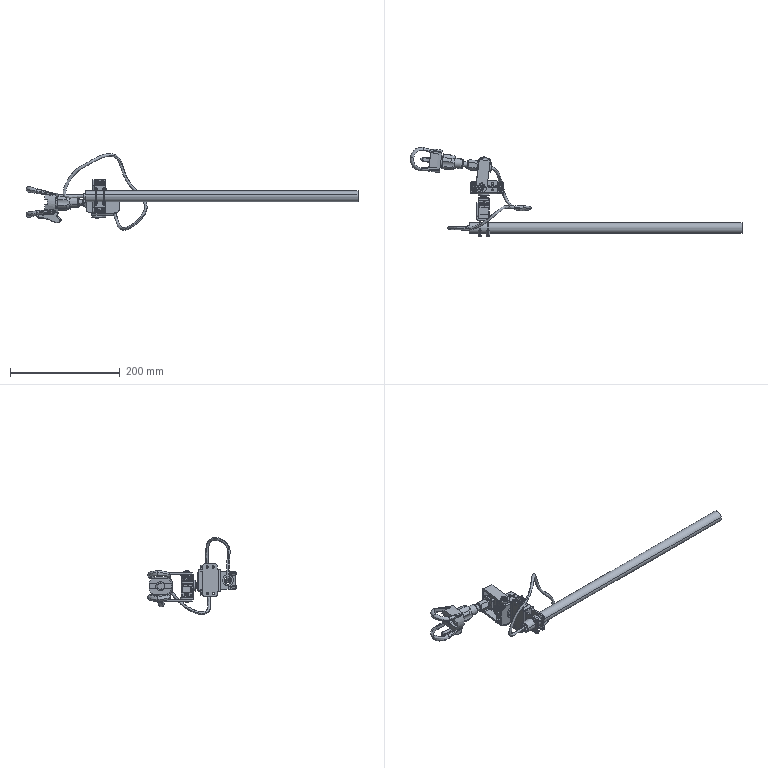Assembly | SolidWorks | mm | 51 component files | 71 solids | 2175 faces | box 605.94 x 162.7 x 140.31 mm | volume 236040 mm3 | plane 965 | cylinder 769 | spline 185 | cone 184 | torus 70 | sphere 2 | commonest cylinder face diameters 0.4 x120 2 x91 1.5 x64 3.5 x58 4 x55 6 x36 1 x32 3 x30
Bill of materials:
Bracket | 1 | 45 | Folded plate bracket. A flat web has two parallel flanges bent at right angles from opposite ends, each with two through holes. A second offset plate section carries two parallel tabs, and each tab has an open semicircular notch.
Bracket2 | 1 | 45 | Bent plate bracket shaped like an E or a double C. A rectangular back panel with rounded corners joins a perforated top flange. Two narrower ears with holes extend parallel to the top flange.
Bracket3 | 1 | 45 | U-shaped (clevis-like) bracket. A rectangular base web has two long parallel arms with rounded ends. The base web and both arm ends carry radial patterns of round holes.
bzd | 1 |  | Irregular, organically contoured flat body like a paddle or lever. A cylindrical post stands perpendicular to it, and a small coaxial pin sticks out of one narrow end.
Card | 4 | 45 | Rectangular block with a semicircular cutout centred on one long edge. Two small through holes run through the end lugs on either side of the cutout.
cross recessed cheese head screws type a gb | 4 |  | Headed cylindrical pin, similar in form to a pan- or cheese-head screw. It has a cross-shaped recess in the head, a short neck below the head and a plain cylindrical shank.
GB_FASTENER_SCREWS_HSHCS M2X3-N | 4 |  | Short headed pin made of two coaxial cylinders: a larger cylindrical head with rounded outer edge and a shorter, smaller-diameter plain cylindrical shank with chamfered tip. Looks like a cap-head screw with no threads modeled.
GB_FASTENER_SCREWS_HSHCS M3X10-N | 4 |  | Long headed pin: a cylindrical head with rounded outer edge on one end of a long, smaller-diameter plain cylindrical shank with chamfered tip. Looks like a socket-head cap screw with no threads modeled.
GB_FASTENER_SCREWS_HSHCS M4X10-N | 4 |  | Socket-head-style headed pin: a cylindrical head with rounded top edge and a hexagonal recess in the head, plus a smaller-diameter plain cylindrical shank with chamfered tip.
GB_FASTENER_SCREWS_HSHCS M3X6-N | 2 |  | Stepped cylindrical headed pin: a large-diameter cylindrical head with rounded edge and a smaller plain cylindrical shank with chamfered tip, about 1.5-2 times the head height in length.
GB_FASTENER_SCREWS_HSHCS M4X6-N | 1 |  | Short headed pin made of two coaxial cylinders: a cylindrical head with rounded outer edge, a polygonal (likely hex) recess at the head end, and a short smaller-diameter plain cylindrical shank with chamfered tip. Nearly identical to unnamed part.
jiazi1 | 1 |  | Compact block with a central through hole, from which two curved strap or loop arms extend. The arms form an open loop or bail shape.
lumu | 1 |  | Short tubular sleeve with a central bore. The outer profile is lobed or fluted, chamfered toward one end and stepped down to a smaller round diameter at the other end.
MG996RServo_stp | 2 | 45 | Rectangular box-shaped housing. Two mounting ears with open-ended slots project from opposite ends. It has a round output boss with a stepped cylindrical shaft on one face and a small multi-wire cable exit.
Part10 | 2 | 45 | Thick plate with a large semicircular cutout on one long edge. Two cylindrical bosses run along the opposite face at each end, each with a through hole.
Part12 | 1 | 45 | Stepped cylindrical pin. It has a domed tip, two raised collars along the shaft and a larger flanged head at the other end with a shallow recessed face.
Part13 | 1 | 45 | Hexagonal sleeve, like a long hex nut or standoff. It has a round through bore, chamfered hex corners at both ends and a short round spigot or shoulder at one end.
Part5 | 1 | 45 | Solid straight cylindrical rod with plain flat ends.
Part6 | 1 | 45 | Circular flange disc with a smaller concentric cylindrical hub on one face. It has a central through bore and three smaller round through holes spaced around the lower part of the bore. The lowest small hole appears to break into the hub's edge and leave a notch.
Part7 | 1 | 45 | Short solid cylinder, about as long as it is wide, with an obround (slot-shaped) opening in one flat end that runs along the axis.
Part9 | 1 | 45 | Long, thin, straight round tube (hollow cylinder) with open, square-cut ends.
plain washers-n series-grade a gb | 2 |  | Flat circular ring (washer-like annulus) with a concentric through hole and parallel flat faces.
prevailing torque all-metal 1 gb M4 | 4 |  | Hexagonal prism with a plain central round through bore. Both ends have a conical edge chamfer, which shows as curved arcs on each flat face, and the axial length is relatively long.
prevailing torque all-metal 1 gb | 4 |  | Hexagonal prism with a central round through bore, chamfered corners at both ends, and a countersink or chamfer at the bore entrance. It is shorter than it is wide across the corners.
White | 1 |  | Stepped solid shaft or pin made of three coaxial cylindrical sections: a large plain section, a slightly larger middle section with a chamfer at its outer end, and a much smaller pin projecting from the chamfered end with a flat tip.
Wire | 1 | 45 | Thin round wire or flexible tube bent along an irregular, freeform three-dimensional path with two free open ends.
Mates:
1. coincident | MG996RServo_stp-1 plane at (0, 0, 0) dir (0, 0, 1) | assembly plane at (0, 0, 0) dir (0, 0, 1)
2. coincident | MG996RServo_stp-1 plane at (0, 0, 0) dir (0, 1, 0) | assembly plane at (0, 0, 0) dir (0, 1, 0)
3. coincident | MG996RServo_stp-1 plane at (0, 0, 0) dir (1, 0, 0) | assembly plane at (0, 0, 0) dir (1, 0, 0)
4. concentric | MG996RServo_stp-1 face at (0, 69.1, 0) dir (0, -1, 0) r 2.97 | Part6-1 face at (0, 15.25, 0) dir (0, -1, 0) r 3
5. coincident | MG996RServo_stp-1 face at (0, 12.25, 0) dir (0, 1, 0) | Part6-1 face at (0, 12.25, 0) dir (0, -1, 0)
6. coincident | Bracket2-1 face at (-14.529, 17.25, 0.1423) dir (-1, 0, 0.009793) | MG996RServo_stp-3 face at (-14.66, 20.493, -13.203) dir (-1, 0, 0.009793)
7. coincident | Bracket2-1 face at (25.255, 42.25, -22.094) dir (0.009793, 0, 1) | MG996RServo_stp-3 face at (-4.743, 30.493, -21.8) dir (-0.009793, 0, -1)
8. coincident | Bracket-1 face at (0, -45, 0) dir (0, -1, 0) | Part10-2 face at (-8.904, -45, -6.496) dir (0, 1, 0)
9. coincident | Bracket-1 face at (-5.904, -45, 26.504) dir (1, 0, 0) | Part10-2 face at (-5.904, -45, 10.004) dir (1, 0, 0)
10. coincident | Bracket-1 face at (-5.904, -45, -6.496) dir (0, 0, -1) | Part10-2 face at (-8.904, -59.182, -6.496) dir (0, 0, -1)
11. concentric | Bracket2-1 edge at (-4.322, 30.493, 21.197) dir (0.009793, 0, 1) r 3.1 | Bracket3-1 face at (-4.288, 30.493, 24.697) dir (-0.009793, 0, -1) r 1.75
12. coincident | Bracket2-1 face at (25.676, 17.25, 20.904) dir (0.009793, 0, 1) | Bracket3-1 face at (4.424, 19.38, 21.112) dir (-0.009793, 0, -1)
13. concentric | Bracket3-1 face at (5.102, 60.069, 6.604) dir (0.1183, 0.993, -0.001159) r 1 | Card-1 face at (5.871, 66.524, 6.597) dir (0.1183, 0.993, -0.001159) r 0.75
14. concentric | Bracket3-1 face at (4.936, 60.069, -10.395) dir (0.1183, 0.993, -0.001159) r 1 | Card-1 face at (5.705, 66.524, -10.402) dir (0.1183, 0.993, -0.001159) r 0.75
15. coincident | Bracket3-1 face at (10.717, 75.98, -24.952) dir (-0.1183, -0.993, 0.001159) | Card-1 face at (5.131, 76.66, -12.397) dir (0.1183, 0.993, -0.001159)
16. coincident | Card-1 face at (7.423, 66.316, -12.419) dir (0.9929, -0.1183, -0.009724) | Card-2 face at (7.423, 66.316, -12.419) dir (0.9929, -0.1183, -0.009724)
17. coincident | Card-1 edge at (5.705, 66.524, -10.402) dir (0.1183, 0.993, -0.001159) r 0.75 | Card-2 edge at (5.705, 66.524, -10.402) dir (-0.1183, -0.993, 0.001159) r 0.75
18. concentric | Bracket3-1 edge at (-4.613, 81.349, -10.301) dir (0.1183, 0.993, -0.001159) r 1 | Card-3 edge at (-5.027, 77.873, -10.297) dir (0.1183, 0.993, -0.001159) r 0.75
19. concentric | Bracket3-1 face at (-6.813, 61.489, 6.721) dir (0.1183, 0.993, -0.001159) r 1 | Card-3 face at (-6.044, 67.943, 6.714) dir (0.1183, 0.993, -0.001159) r 0.75
20. coincident | Bracket3-1 face at (10.717, 75.98, -24.952) dir (-0.1183, -0.993, 0.001159) | Card-3 face at (-6.785, 78.08, -12.28) dir (0.1183, 0.993, -0.001159)
21. coincident | Card-3 face at (-7.968, 68.151, -12.268) dir (-0.9929, 0.1183, 0.009724) | Card-4 face at (-7.968, 68.151, -12.268) dir (-0.9929, 0.1183, 0.009724)
22. coincident | Card-3 face at (-8.323, 65.172, -12.265) dir (-0.009793, 0, -1) | Card-4 face at (-4.138, 70.715, -12.306) dir (-0.009793, 0, -1)
23. coincident | Card-3 face at (-7.968, 68.151, -12.268) dir (-0.1183, -0.993, 0.001159) | Card-4 face at (-4.493, 67.736, -12.302) dir (0.1183, 0.993, -0.001159)
24. concentric | Bracket-1 edge at (-8.904, -45, 10.004) dir (-1, 0, 0) r 10 | Part9-1 face at (-27.046, -45, 10.004) dir (1, 0, 0) r 10
25. distance | Bracket-1 face at (5.904, -45, 26.504) dir (-1, 0, 0) | Part9-1 face at (-27.046, -45, 10.004) dir (-1, 0, 0)
26. concentric | Part9-1 face at (470.954, -45, 10.004) dir (-1, 0, 0) r 7 | Part5-1 face at (-29.297, -45, 10.004) dir (-1, 0, 0) r 4.5
27. concentric | Bracket3-1 face at (-6.98, 61.489, -10.278) dir (0.1183, 0.993, -0.001159) r 1 | hexagon socket head cap screws gb-1 face at (-4.968, 78.37, -10.298) dir (0.1183, 0.993, -0.001159) r 1
28. coincident | Bracket3-1 face at (11.616, 79.455, 24.542) dir (0.1183, 0.993, -0.001159) | hexagon socket head cap screws gb-1 face at (-4.613, 81.349, -10.301) dir (-0.1183, -0.993, 0.001159)
29. concentric | Bracket3-1 face at (-6.813, 61.489, 6.721) dir (0.1183, 0.993, -0.001159) r 1 | hexagon socket head cap screws gb-2 face at (-4.802, 78.37, 6.701) dir (0.1183, 0.993, -0.001159) r 1
30. coincident | Bracket3-1 face at (11.616, 79.455, 24.542) dir (0.1183, 0.993, -0.001159) | hexagon socket head cap screws gb-2 face at (-4.447, 81.349, 6.698) dir (-0.1183, -0.993, 0.001159)
31. concentric | Bracket3-1 face at (5.102, 60.069, 6.604) dir (0.1183, 0.993, -0.001159) r 1 | hexagon socket head cap screws gb-3 face at (7.113, 76.95, 6.585) dir (0.1183, 0.993, -0.001159) r 1
32. coincident | Bracket3-1 face at (11.616, 79.455, 24.542) dir (0.1183, 0.993, -0.001159) | hexagon socket head cap screws gb-3 face at (7.468, 79.929, 6.581) dir (-0.1183, -0.993, 0.001159)
33. concentric | Bracket3-1 face at (4.936, 60.069, -10.395) dir (0.1183, 0.993, -0.001159) r 1 | hexagon socket head cap screws gb-4 face at (6.947, 76.95, -10.414) dir (0.1183, 0.993, -0.001159) r 1
34. coincident | Bracket3-1 face at (11.616, 79.455, 24.542) dir (0.1183, 0.993, -0.001159) | hexagon socket head cap screws gb-4 face at (7.302, 79.929, -10.418) dir (-0.1183, -0.993, 0.001159)
35. concentric | Bracket3-1 face at (-0.9388, 60.779, -1.837) dir (0.1183, 0.993, -0.001159) r 2.5 | hexagon socket head cap screws gb-5 face at (0.7177, 74.681, -1.853) dir (0.1183, 0.993, -0.001159) r 2
36. coincident | Bracket3-1 face at (11.616, 79.455, 24.542) dir (0.1183, 0.993, -0.001159) | hexagon socket head cap screws gb-5 face at (1.428, 80.639, -1.86) dir (-0.1183, -0.993, 0.001159)
37. concentric | MG996RServo_stp-1 face at (5, -6.364, -14.25) dir (0, 1, 0) r 2.25 | hexagon socket head cap screws gb-10 face at (5, -7.6, -14.25) dir (0, 1, 0) r 1.5
38. coincident | MG996RServo_stp-1 face at (0, 2.4, 0) dir (0, 1, 0) | hexagon socket head cap screws gb-10 face at (5, 2.4, -14.25) dir (0, -1, 0)
39. concentric | MG996RServo_stp-1 face at (-5, -6.364, -14.25) dir (0, 1, 0) r 2.25 | hexagon socket head cap screws gb-11 face at (-5, -7.6, -14.25) dir (0, 1, 0) r 1.5
40. coincident | MG996RServo_stp-1 face at (0, 2.4, 0) dir (0, 1, 0) | hexagon socket head cap screws gb-11 face at (-5, 2.4, -14.25) dir (0, -1, 0)
41. concentric | MG996RServo_stp-1 face at (5, -6.364, 34.25) dir (0, 1, 0) r 2.25 | hexagon socket head cap screws gb-12 face at (5, -7.6, 34.25) dir (0, 1, 0) r 1.5
42. coincident | MG996RServo_stp-1 face at (0, 2.4, 0) dir (0, 1, 0) | hexagon socket head cap screws gb-12 face at (5, 2.4, 34.25) dir (0, -1, 0)
43. concentric | MG996RServo_stp-1 face at (-5, -6.364, 34.25) dir (0, 1, 0) r 2.25 | hexagon socket head cap screws gb-13 face at (-5, -7.6, 34.25) dir (0, 1, 0) r 1.5
44. coincident | MG996RServo_stp-1 face at (0, 2.4, 0) dir (0, 1, 0) | hexagon socket head cap screws gb-13 face at (-5, 2.4, 34.25) dir (0, -1, 0)
45. concentric | Part10-1 face at (7.404, -45, 22.004) dir (0, -1, 0) r 0.75 | cross recessed cheese head screws type a gb-1 face at (7.404, -58.182, 22.004) dir (0, -1, 0) r 104.72
46. coincident | Part10-1 face at (5.904, -59.182, 26.504) dir (0, -1, 0) | cross recessed cheese head screws type a gb-1 face at (7.404, -59.182, 22.004) dir (0, 1, 0)
47. concentric | Part10-2 face at (-7.404, -45, 22.004) dir (0, -1, 0) r 0.75 | cross recessed cheese head screws type a gb-2 face at (-7.404, -58.182, 22.004) dir (0, -1, 0) r 104.72
48. coincident | Part10-2 face at (-8.904, -59.182, 26.504) dir (0, -1, 0) | cross recessed cheese head screws type a gb-2 face at (-7.404, -59.182, 22.004) dir (0, 1, 0)
49. concentric | Part10-2 face at (-7.404, -45, -1.996) dir (0, -1, 0) r 0.75 | cross recessed cheese head screws type a gb-3 face at (-7.404, -58.182, -1.996) dir (0, -1, 0) r 104.72
50. coincident | Part10-2 face at (-8.904, -59.182, 26.504) dir (0, -1, 0) | cross recessed cheese head screws type a gb-3 face at (-7.404, -59.182, -1.996) dir (0, 1, 0)
51. concentric | Part10-1 face at (7.404, -45, -1.996) dir (0, -1, 0) r 0.75 | cross recessed cheese head screws type a gb-4 face at (7.404, -58.182, -1.996) dir (0, -1, 0) r 104.72
52. coincident | Part10-1 face at (5.904, -59.182, 26.504) dir (0, -1, 0) | cross recessed cheese head screws type a gb-4 face at (7.404, -59.182, -1.996) dir (0, 1, 0)
53. concentric | MG996RServo_stp-3 face at (-18.776, 35.493, 0.4741) dir (0.009793, 0, 1) r 2.25 | hexagon socket head cap screws gb-14 face at (-18.788, 35.493, -0.7619) dir (0.009793, 0, 1) r 2
54. coincident | MG996RServo_stp-3 face at (-4.441, 30.493, 9.098) dir (0.009793, 0, 1) | hexagon socket head cap screws gb-14 face at (-18.69, 35.493, 9.238) dir (-0.009793, 0, -1)
55. concentric | MG996RServo_stp-3 face at (-18.776, 25.493, 0.4741) dir (0.009793, 0, 1) r 2.25 | hexagon socket head cap screws gb-15 face at (-18.788, 25.493, -0.7619) dir (0.009793, 0, 1) r 2
56. coincident | MG996RServo_stp-3 face at (-4.441, 30.493, 9.098) dir (0.009793, 0, 1) | hexagon socket head cap screws gb-15 face at (-18.69, 25.493, 9.238) dir (-0.009793, 0, -1)
57. concentric | MG996RServo_stp-3 face at (29.722, 35.493, -0.0009) dir (0.009793, 0, 1) r 2.25 | hexagon socket head cap screws gb-16 face at (29.71, 35.493, -1.237) dir (0.009793, 0, 1) r 2
58. coincident | MG996RServo_stp-3 face at (-4.441, 30.493, 9.098) dir (0.009793, 0, 1) | hexagon socket head cap screws gb-16 face at (29.808, 35.493, 8.763) dir (-0.009793, 0, -1)
59. concentric | MG996RServo_stp-3 face at (29.722, 25.493, -0.0009) dir (0.009793, 0, 1) r 2.25 | hexagon socket head cap screws gb-17 face at (29.71, 25.493, -1.237) dir (0.009793, 0, 1) r 2
60. coincident | MG996RServo_stp-3 face at (-4.441, 30.493, 9.098) dir (0.009793, 0, 1) | hexagon socket head cap screws gb-17 face at (29.808, 25.493, 8.763) dir (-0.009793, 0, -1)
61. concentric | Bracket3-1 face at (-4.288, 30.493, 24.697) dir (-0.009793, 0, -1) r 1.75 | plain washers-n series-grade a gb-1 face at (-4.288, 30.493, 24.697) dir (0.009793, 0, 1) r 2.75
62. coincident | Bracket3-1 face at (4.458, 19.38, 24.612) dir (0.009793, 0, 1) | plain washers-n series-grade a gb-1 face at (-4.288, 30.493, 24.697) dir (-0.009793, 0, -1)
63. concentric | Bracket3-1 face at (-4.288, 30.493, 24.697) dir (-0.009793, 0, -1) r 1.75 | plain washers-n series-grade a gb-3 face at (-4.807, 30.493, -28.3) dir (-0.009793, 0, -1) r 2.75
64. coincident | Bracket3-1 face at (3.939, 19.38, -28.386) dir (-0.009793, 0, -1) | plain washers-n series-grade a gb-3 face at (-4.807, 30.493, -28.3) dir (0.009793, 0, 1)
65. concentric | Bracket3-1 face at (-4.288, 30.493, 24.697) dir (-0.009793, 0, -1) r 1.75 | hexagon socket head cap screws gb-19 face at (-4.748, 30.493, -22.3) dir (-0.009793, 0, -1) r 1.5
66. coincident | Bracket3-1 face at (3.939, 19.38, -28.386) dir (-0.009793, 0, -1) | hexagon socket head cap screws gb-19 face at (-4.807, 30.493, -28.3) dir (0.009793, 0, 1)
67. concentric | Bracket3-1 face at (-4.288, 30.493, 24.697) dir (-0.009793, 0, -1) r 1.75 | hexagon socket head cap screws gb-20 face at (-4.347, 30.493, 18.698) dir (0.009793, 0, 1) r 1.5
68. coincident | Bracket3-1 face at (4.458, 19.38, 24.612) dir (0.009793, 0, 1) | hexagon socket head cap screws gb-20 face at (-4.288, 30.493, 24.697) dir (-0.009793, 0, -1)
69. concentric | hexagon socket head cap screws gb-11 face at (-5, -7.6, -14.25) dir (0, 1, 0) r 1.5 | prevailing torque all-metal 1 gb-1 face at (-5, -8.3, -14.25) dir (0, 1, 0) r 1.7
70. concentric | hexagon socket head cap screws gb-10 face at (5, -7.6, -14.25) dir (0, 1, 0) r 1.5 | prevailing torque all-metal 1 gb-2 face at (5, -8.3, -14.25) dir (0, 1, 0) r 1.7
71. concentric | hexagon socket head cap screws gb-13 face at (-5, -7.6, 34.25) dir (0, 1, 0) r 1.5 | prevailing torque all-metal 1 gb-3 face at (-5, -8.3, 34.25) dir (0, 1, 0) r 1.7
72. concentric | hexagon socket head cap screws gb-12 face at (5, -7.6, 34.25) dir (0, 1, 0) r 1.5 | prevailing torque all-metal 1 gb-4 face at (5, -8.3, 34.25) dir (0, 1, 0) r 1.7
73. concentric | hexagon socket head cap screws gb-16 face at (29.71, 35.493, -1.237) dir (0.009793, 0, 1) r 2 | prevailing torque all-metal 1 gb M4-5 face at (29.698, 35.493, -2.437) dir (0.009793, 0, 1) r 2
74. concentric | hexagon socket head cap screws gb-17 face at (29.71, 25.493, -1.237) dir (0.009793, 0, 1) r 2 | prevailing torque all-metal 1 gb M4-6 face at (29.698, 25.493, -2.437) dir (0.009793, 0, 1) r 2
75. concentric | hexagon socket head cap screws gb-14 face at (-18.788, 35.493, -0.7619) dir (0.009793, 0, 1) r 2 | prevailing torque all-metal 1 gb M4-7 face at (-18.8, 35.493, -1.962) dir (0.009793, 0, 1) r 2
76. concentric | hexagon socket head cap screws gb-15 face at (-18.788, 25.493, -0.7619) dir (0.009793, 0, 1) r 2 | prevailing torque all-metal 1 gb M4-8 face at (-18.8, 25.493, -1.962) dir (0.009793, 0, 1) r 2
77. coincident | Bracket2-1 face at (25.416, 40.25, 2.905) dir (-0.009793, 0, -1) | prevailing torque all-metal 1 gb M4-5 face at (25.75, 33.184, 2.902) dir (0.009793, 0, 1)
78. coincident | Bracket2-1 face at (25.416, 40.25, 2.905) dir (-0.009793, 0, -1) | prevailing torque all-metal 1 gb M4-6 face at (25.75, 23.184, 2.902) dir (0.009793, 0, 1)
79. coincident | Bracket2-1 face at (-14.498, 40.25, 3.296) dir (-0.009793, 0, -1) | prevailing torque all-metal 1 gb M4-7 face at (-22.748, 33.184, 3.377) dir (0.009793, 0, 1)
80. coincident | Bracket2-1 face at (-14.498, 40.25, 3.296) dir (-0.009793, 0, -1) | prevailing torque all-metal 1 gb M4-8 face at (-22.748, 23.184, 3.377) dir (0.009793, 0, 1)
81. concentric | Part13-1 face at (-29.213, 70.695, -1.56) dir (0.9929, -0.1183, -0.009724) r 5 | White-1 face at (-38.038, 71.746, -1.473) dir (0.9929, -0.1183, -0.009724) r 5
82. coincident | Part12-1 edge at (-29.102, 70.681, -1.561) dir (0.9929, -0.1183, -0.009724) r 1 | White-1 face at (-29.102, 70.681, -1.561) dir (0.9929, -0.1183, -0.009724)
83. concentric | White-1 face at (-53.925, 73.639, -1.318) dir (-0.9929, 0.1183, 0.009724) r 8.34 | lumu-1 face at (-78.748, 76.598, -1.075) dir (0.9929, -0.1183, -0.009724) r 8.34
84. coincident | White-1 face at (-53.925, 73.639, -1.318) dir (-0.9929, 0.1183, 0.009724) | lumu-1 face at (-53.925, 73.639, -1.318) dir (0.9929, -0.1183, -0.009724)
85. concentric | lumu-1 face at (-78.748, 76.598, -1.075) dir (0.9929, -0.1183, -0.009724) r 8.34 | jiazi1-1 face at (-98.607, 78.964, -0.8802) dir (0.9929, -0.1183, -0.009724) r 8.34
86. coincident | lumu-1 face at (-78.748, 76.598, -1.075) dir (-0.9929, 0.1183, 0.009724) | jiazi1-1 face at (-78.748, 76.598, -1.075) dir (0.9929, -0.1183, -0.009724)
87. concentric | jiazi1-1 face at (-86.725, 77.525, -20.998) dir (0.009793, 0, 1) r 3.8 | bzd-1 face at (-86.895, 77.525, -38.414) dir (0.009793, 0, 1) r 3.8
88. parallel | jiazi1-1 face at (-98.607, 78.964, -0.8802) dir (-0.9929, 0.1183, 0.009724) | bzd-1 face at (-115.572, 80.956, -26.049) dir (-0.9929, 0.1183, 0.009724)
89. coincident | jiazi1-1 face at (-90.215, 107.544, -5.963) dir (0.009793, 0, 1) | bzd-1 face at (-86.578, 77.525, -5.998) dir (0.009793, 0, 1)
90. parallel | Bracket3-1 face at (3.939, 19.38, -28.386) dir (-0.009793, 0, -1) | jiazi1-1 face at (-90.117, 107.544, 4.037) dir (-0.009793, 0, -1)
91. parallel | Bracket3-1 face at (3.939, 19.38, -28.386) dir (-0.009793, 0, -1) | lumu-1 plane at (-53.925, 73.639, -1.318) dir (-0.009793, 0, -1)
92. coincident | Bracket-1 face at (10.404, -3, -9.907) dir (0, -1, 0) | prevailing torque all-metal 1 gb-1 face at (-7.519, -3, -10.378) dir (0, 1, 0)
93. coincident | Bracket-1 face at (10.404, -3, -9.907) dir (0, -1, 0) | prevailing torque all-metal 1 gb-2 face at (2.628, -3, -10.287) dir (0, 1, 0)
94. coincident | Bracket-1 face at (10.404, -3, 29.915) dir (0, -1, 0) | prevailing torque all-metal 1 gb-3 face at (-7.159, -3, 38.333) dir (0, 1, 0)
95. coincident | Bracket-1 face at (10.404, -3, 29.915) dir (0, -1, 0) | prevailing torque all-metal 1 gb-4 face at (2.716, -3, 38.265) dir (0, 1, 0)
96. distance | Bracket2-1 face at (0, 20.25, 0) dir (0, 1, 0) | MG996RServo_stp-3 face at (-14.66, 20.493, -13.203) dir (0, -1, 0)